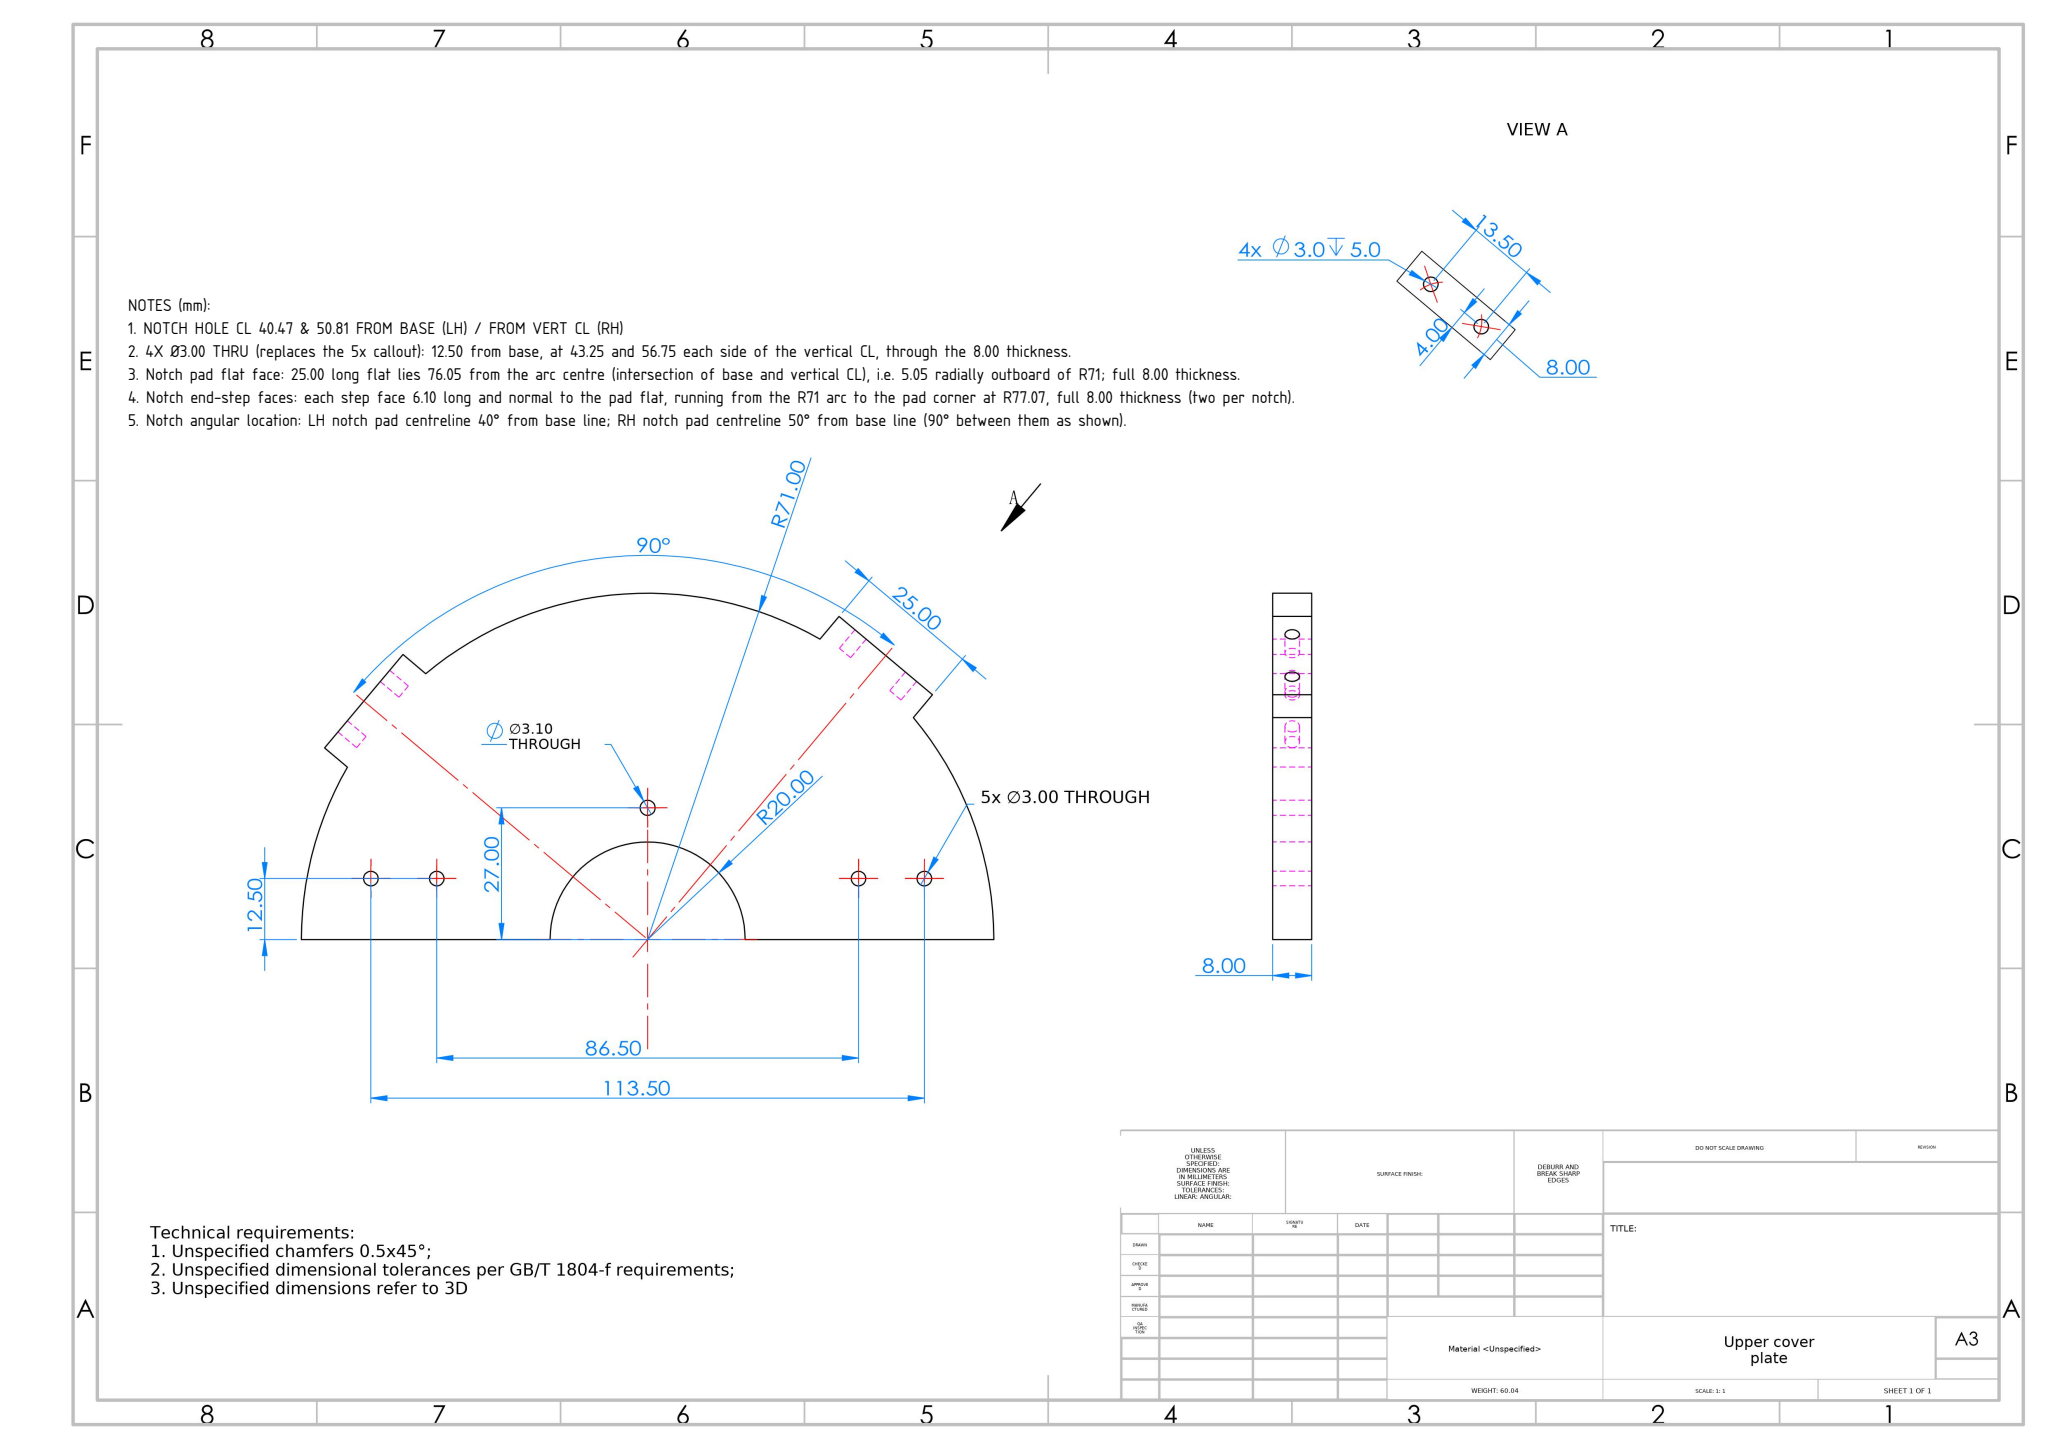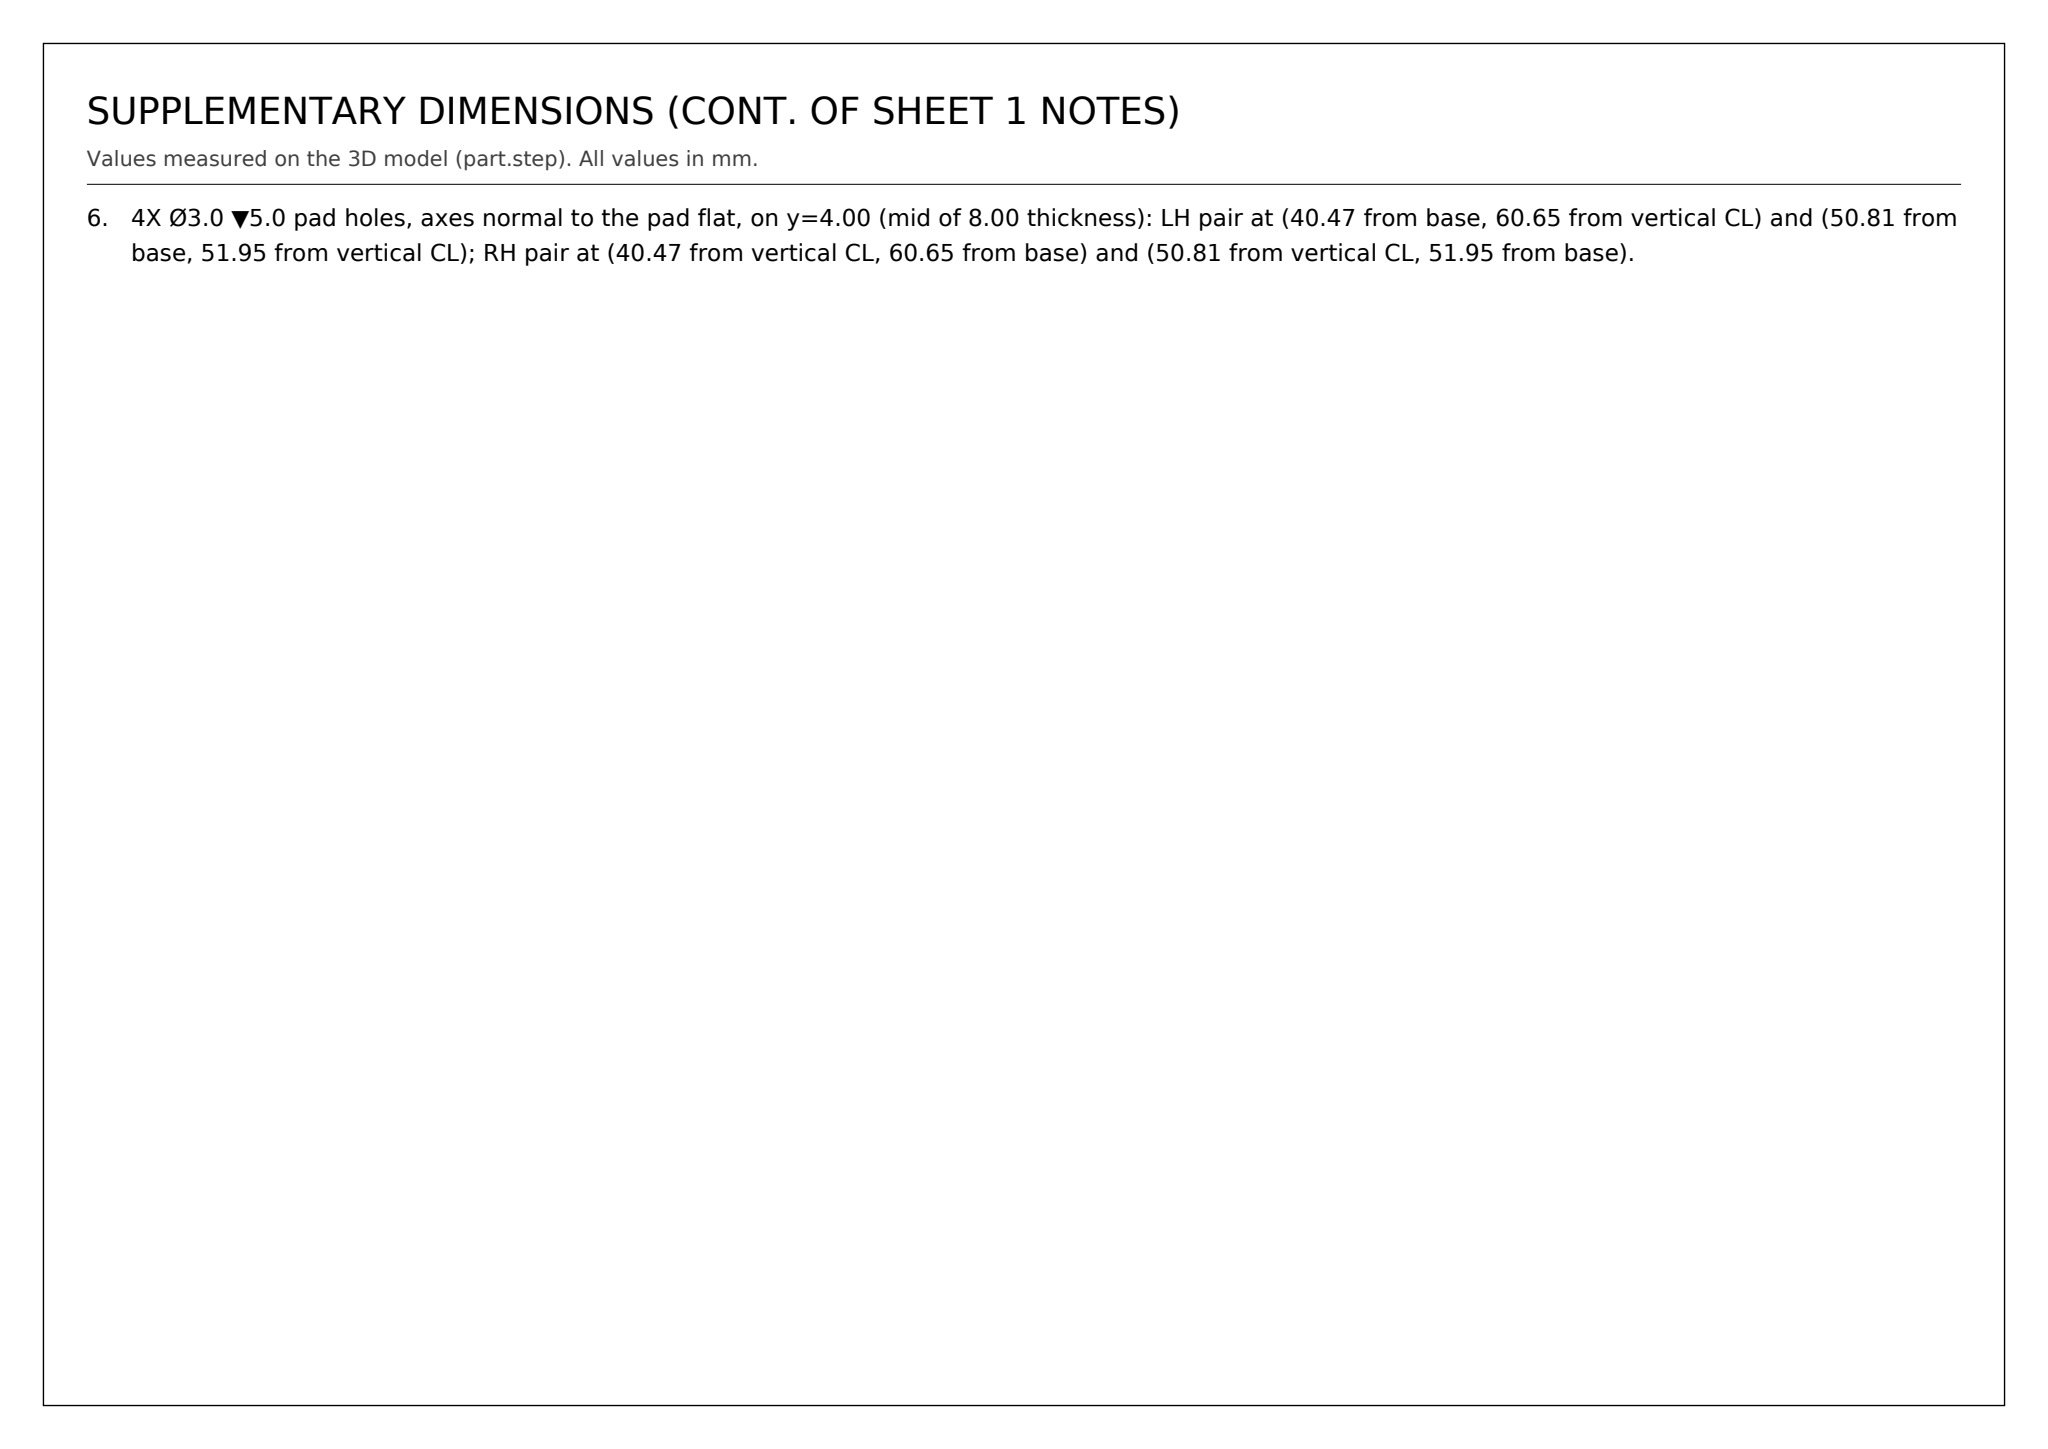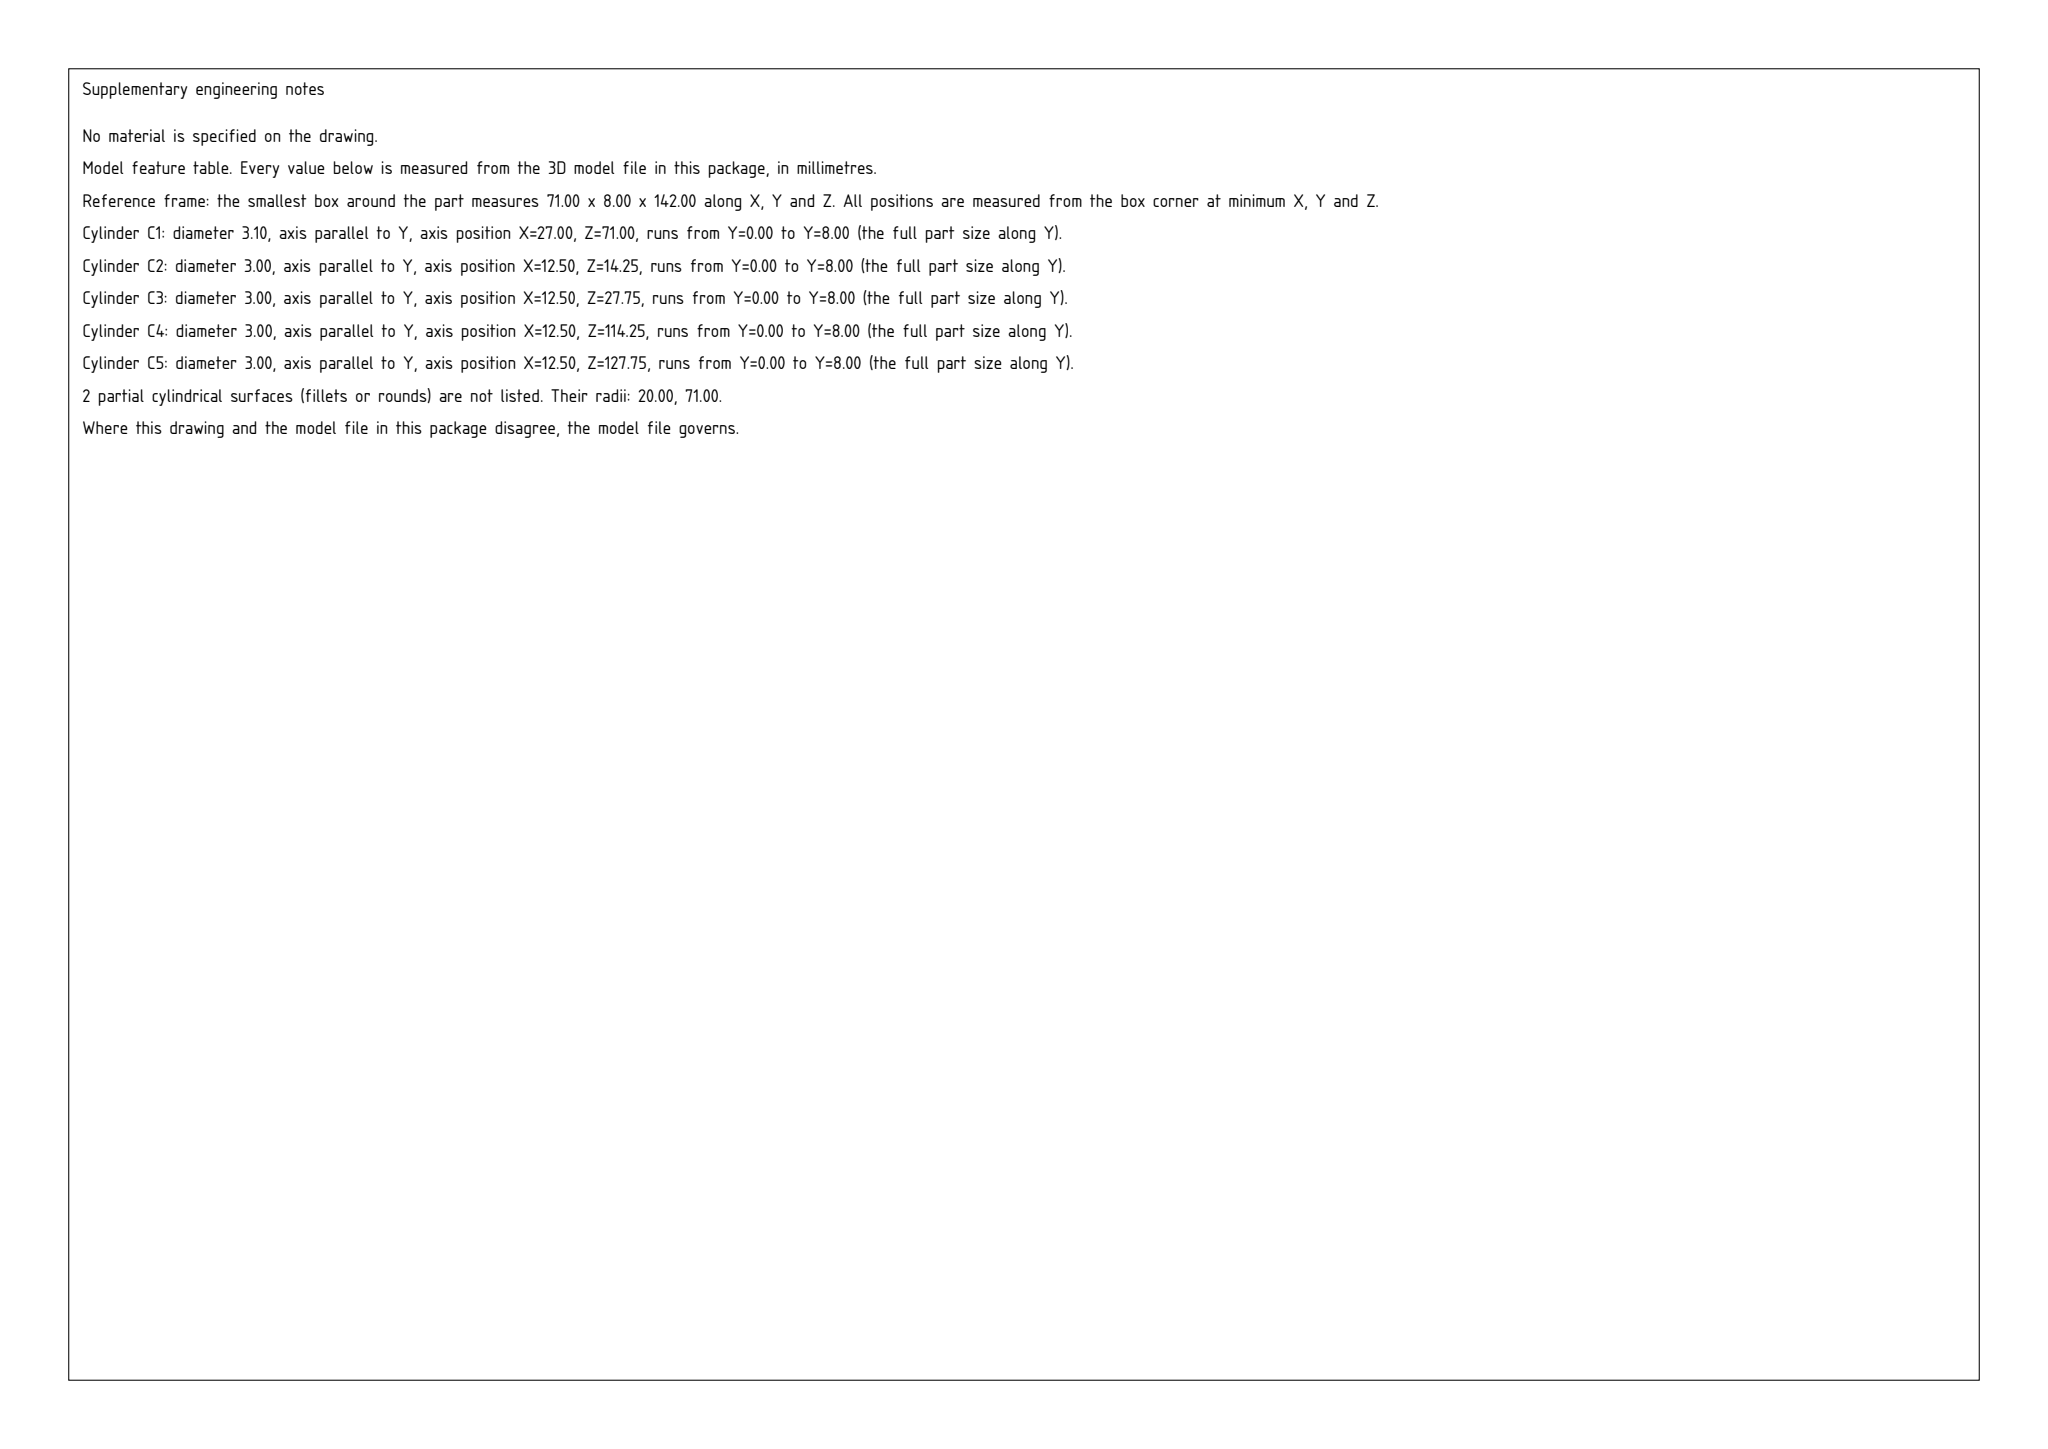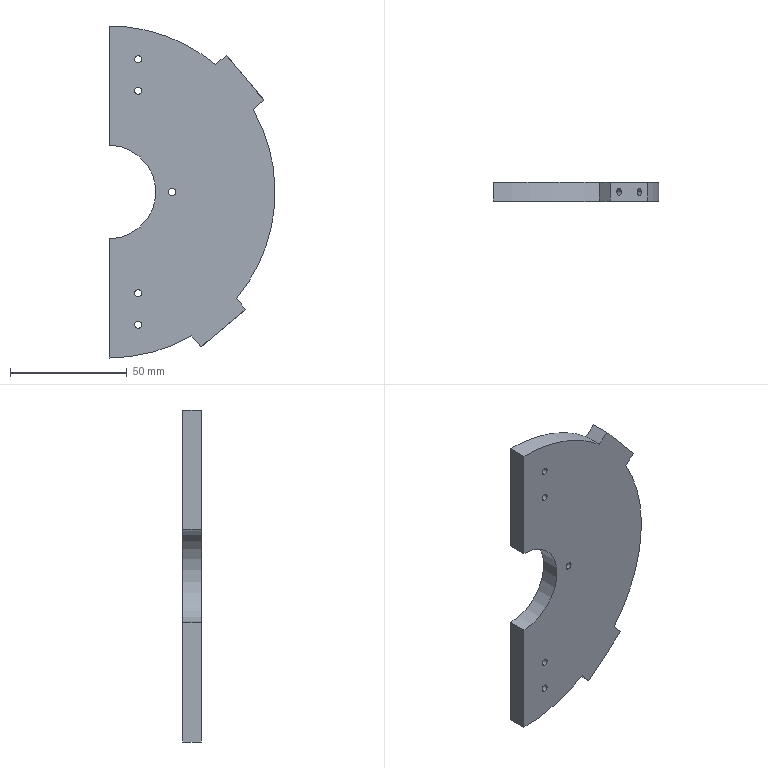Part | SolidWorks | mm | 1 solid | 36 faces | box 71 x 8 x 142 mm | volume 60040 mm3 | cylinder 22 | plane 14 | commonest cylinder face diameters 3 x16 142 x3 3.1 x2 40 x1
Drawing notes:
NOTCH HOLE CL 40.47 & 50.81 FROM BASE (LH) / FROM VERT CL (RH) | from the solid: axis-z holes x=40.47, 50.81 from plane x=0 (flat base); axis-x holes z=111.47, 121.81 = 40.47 & 50.81 from CL z=71
4X Ø3.00 THRU (replaces the 5x callout): 12.50 from base, at 43.25 and 56.75 each side of the vertical CL, through the 8.00 thickness. | from the solid: cylinders: four 'hole/bore' dia 3.0, axis y, at (x=12.5, z=14.3 / 27.8 / 114.3 / 127.8), from 0.0 to 8.0; plus one separate dia 3.1 at (x=27.0, z=71.0)
Notch pad flat face: 25.00 long flat lies 76.05 from the arc centre (intersection of base and vertical CL), i.e. 5.05 radially outboard of R71; full 8.00 thickness. | from the solid: inclined_planes at bbox_from [39.3,0,4.7] size 19.2x8x16.1 and [50.2,0,110.3] size 16.1x8x19.2 (trace length 25.06, perpendicular distance 76.05 from arc axis at x=0,z=71 of the dia 142 convex arc)
Notch end-step faces: each step face 6.10 long and normal to the pad flat, running from the R71 arc to the pad corner at R77.07, full 8.00 thickness (two per notch). | from the solid: inclined_planes [35.3,0,4.7] & [54.5,0,20.8] size 3.9x8x4.7 and [45.5,0,125.5] & [61.6,0,106.3] size 4.7x8x3.9 (trace 6.10, endpoints at radius 71.0 and 77.07 from arc axis)
Notch angular location: LH notch pad centreline 40° from base line; RH notch pad centreline 50° from base line (90° between them as shown). | from the solid: inclined_planes angle_to_xyz_axes [40,90,50] (LH set) and [50,90,40] (RH set); pad flat midpoints at (x=48.9,z=12.75) and (x=58.25,z=119.9) relative to arc axis x=0,z=71
4X Ø3.0 ▼5.0 pad holes, axes normal to the pad flat, on y=4.00 (mid of 8.00 thickness): LH pair at (40.47 from base, 60.65 from vertical CL) and (50.81 from base, 51.95 from vertical CL); RH pair at (40.47 from vertical CL, 60.65 from base) and (50.81 from vertical CL, 51.95 from base). | from the solid: cylinders dia 3.0 inclined: [40.5,4.0,null] z 7.5-13.2; [50.8,4.0,null] z 16.2-21.9; [null,4.0,111.5] x 57.8-63.5; [null,4.0,121.8] x 49.1-54.8 (axis midpoints: z=10.35, 19.05; x=60.65, 51.95; bbox z range 0-142 so CL at z=71)